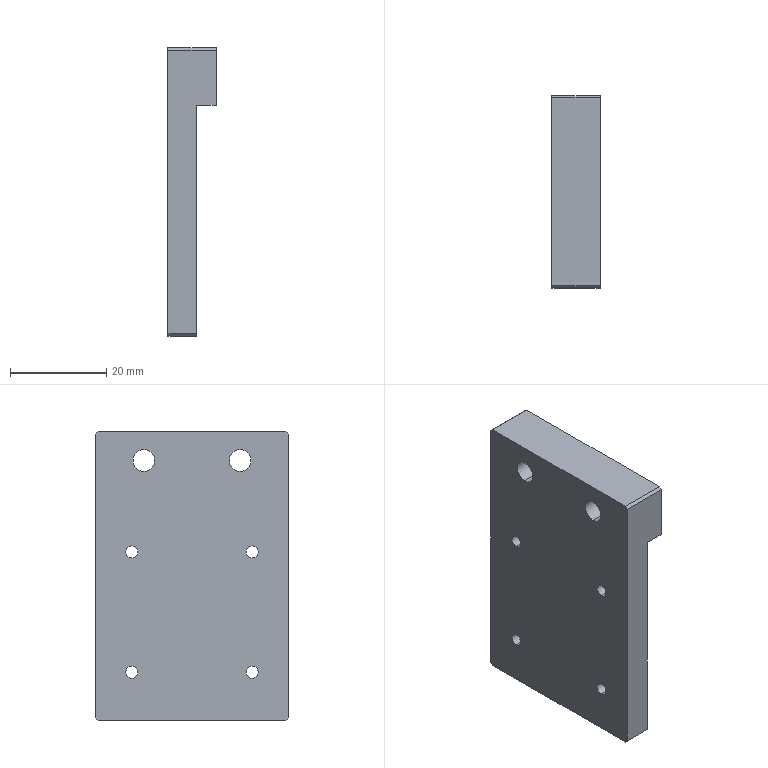Component | SolidWorks | X003.02-011(1)-014-2 | 1 solid | 24 faces | box 10 x 40 x 60 mm | volume 15880 mm3 | cylinder 12 | plane 12 | commonest cylinder face diameters 2.5 x8 4.5 x4 | material AL6061
build123d program:
from build123d import *

# Parameters (mm, degrees)
SKETCH1_W                      = 60
SKETCH1_H                      = 40
BOSS_EXTRUDE1_DEPTH            = 10
SKETCH2_W                      = 48
SKETCH2_H                      = 40
CUT_EXTRUDE1_DEPTH             = 4
CHAMFER1_SIZE                  = 0.5
F_4_5_4_5_DIAMETER_HOLE1_D     = 4.5
F_4_5_4_5_DIAMETER_HOLE1_DEPTH = 15
F_4_5_4_5_DIAMETER_HOLE1_TIP   = 1.352
M3_TAPPED_HOLE1_D              = 2.5
M3_TAPPED_HOLE1_DEPTH          = 7.5
M3_TAPPED_HOLE1_TIP            = 0.7511


with BuildPart() as part:
    # Sketch1 → Boss-Extrude1 (new body)
    with BuildSketch(Plane.XY):
        Rectangle(SKETCH1_W, SKETCH1_H)
    extrude(amount=BOSS_EXTRUDE1_DEPTH)

    # Sketch2 → Cut-Extrude1 (cut)
    with BuildSketch(Plane.XY.offset(10)):
        with Locations((6, 0)):
            Rectangle(SKETCH2_W, SKETCH2_H)
    extrude(amount=-CUT_EXTRUDE1_DEPTH, mode=Mode.SUBTRACT)

    # Chamfer1
    chamfer1_edges = [part.edges().sort_by_distance(p)[0] for p in [
        (30, -20, 3),
        (30, 20, 3),
        (-30, -20, 5),
        (-30, 20, 5),
    ]]
    chamfer(chamfer1_edges, length=CHAMFER1_SIZE)

    # 4.5 _4.5_ Diameter Hole1
    with Locations(Plane(origin=(0, 0, 0), x_dir=(-1, 0, 0), z_dir=(0, 0, -1))):
        with Locations((24, -10), (24, 10)):
            Hole(F_4_5_4_5_DIAMETER_HOLE1_D / 2, depth=F_4_5_4_5_DIAMETER_HOLE1_DEPTH)
            with Locations((0, 0, -(F_4_5_4_5_DIAMETER_HOLE1_DEPTH + F_4_5_4_5_DIAMETER_HOLE1_TIP / 2))):  # 118° drill point
                Cone(0, F_4_5_4_5_DIAMETER_HOLE1_D / 2, F_4_5_4_5_DIAMETER_HOLE1_TIP, mode=Mode.SUBTRACT)

    # M3 Tapped Hole1
    with Locations(Plane(origin=(0, 0, 0), x_dir=(-1, 0, 0), z_dir=(0, 0, -1))):
        with Locations((5, -12.5), (-20, 12.5), (5, 12.5), (-20, -12.5)):
            Hole(M3_TAPPED_HOLE1_D / 2, depth=M3_TAPPED_HOLE1_DEPTH)
            with Locations((0, 0, -(M3_TAPPED_HOLE1_DEPTH + M3_TAPPED_HOLE1_TIP / 2))):  # 118° drill point
                Cone(0, M3_TAPPED_HOLE1_D / 2, M3_TAPPED_HOLE1_TIP, mode=Mode.SUBTRACT)


solid = part.part

# Placed as in the assembly
solid = solid.moved(Location((-186.455, -306.942, 136.696), (0, 90, 0)))